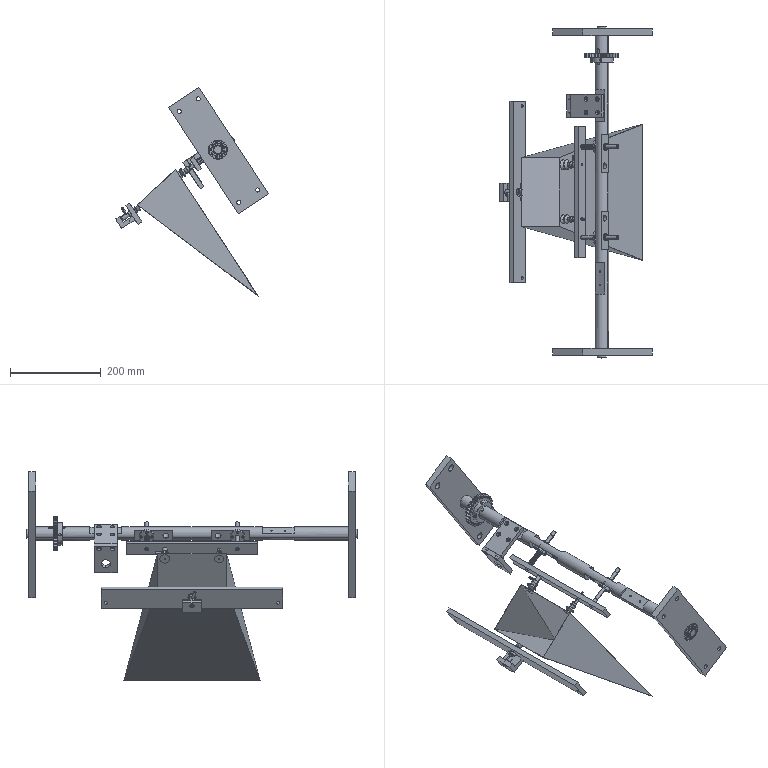Assembly | SolidWorks | mm | 20 component files | 20 solids | 970 faces | box 336.91 x 732 x 460.64 mm | volume 1533403 mm3 | cylinder 371 | plane 217 | sphere 144 | cone 104 | torus 76 | spline 58 | commonest cylinder face diameters 2.5 x32 10 x30 63.75 x29 75 x28 15 x24 6 x19 5 x18 5.5 x18
Bill of materials:
28zGear | 1 |  | Straight-tooth spur gear with a cylindrical hub on one face, a central round bore with a single keyway, and a radial hole through the hub.
BlowOpenBag | 1 |  | Solid tapered wedge or frustum-like block with flat faces only: a rectangular end face that tapers to a narrower edge, giving trapezoidal and triangular outlines in the different views.
CylinderMountingPlate01 | 1 |  | Flat rectangular plate with one large round through hole off-center and two small through holes near one edge.
GB_T276-94DeepGrooveBallBearing6004-2Z | 2 |  | Annular body that looks like a deep-groove ball bearing: an outer ring and an inner ring with a row of balls visible in the gap between them.
HB362-65EndNotTightenedGroundFlat0.25Turns10x50 | 1 | Carbon Spring Steel Wire | Helical coil of round wire with many evenly spaced turns and open, unground-looking ends, like a compression spring.
LMF8UULinearBearing | 2 |  | Flanged cylindrical bushing: a round flange with four equally spaced through holes and a coaxial cylindrical boss with a central through bore.
GuideRod01 | 2 |  | Long slender cylindrical tube with a small coaxial through bore and slightly rounded or chamfered ends.
SuctionCup1 | 1 |  | Body of revolution with two stacked conical bellows-like flares at one end and a stepped cylindrical stem of decreasing diameters, ending in a small tube with a central bore.
SuctionCup2 | 1 |  | Body of revolution like the preceding flared part: two conical bellows-like flares, stepped cylindrical sections and a thicker cylindrical end with a small axial hole, plus a solid pin sticking out sideways near the end.
SuctionCupMountingPlate | 1 |  | Long thin flat rectangular bar with four through holes in a row along its centerline; one hole is larger than the other three.
PullSuctionCupMountingPlate | 1 |  | L-shaped angle bracket of constant thickness with one through hole in one leg and two through holes in the other leg.
ShimPlate02 | 1 |  | Flat rectangular plate with four counterbored through holes in a rectangular pattern, set off to one side of the plate.
SuctionCup3 | 1 |  | Turned body that revolves around one axis. It has a plain cylindrical section, a short step, then several frustum (cone-shaped) and disc-like sections that alternate in direction to give a stepped, waisted profile. It ends in a flat circular face with a small central hole. A slender tube with an open bore branches off the cylindrical section at an angle.
SuctionCupRotatingShaftFixingPlate | 2 | 6061 Alloy | Flat rectangular plate. It has one larger circular hole near the middle and four small round holes, two near each short end, laid out symmetrically.
SupportPlate | 1 |  | Long, thin rectangular bar or plate. It has a larger circular hole at mid-length, two smaller holes beside it that look stepped, and one small hole near each end.
SwingAxis1 | 1 | 45 | Long, slender shaft with steps along its length. Both ends step down to smaller diameters. Several sections in the middle have reduced diameters or flats, and some of those flats have small round cross-holes. Seen end-on, it shows concentric circular steps.
Mates:
1. coincident | SwingAxis1-1 face at (-28.685, 307.546, 10.43) dir (0, 1, 0) | GB_T276-94DeepGrooveBallBearing6004-2Z-1 face at (-15.235, 307.546, 10.43) dir (0, -1, 0)
2. concentric | SwingAxis1-1 face at (-28.685, 325.546, 10.43) dir (0, -1, 0) r 10 | GB_T276-94DeepGrooveBallBearing6004-2Z-1 face at (-28.685, 325.966, 10.43) dir (0, 1, 0) r 10
3. concentric | SwingAxis1-1 face at (-28.685, -406.454, 10.43) dir (0, 1, 0) r 10 | GB_T276-94DeepGrooveBallBearing6004-2Z-2 face at (-28.685, -406.875, 10.43) dir (0, -1, 0) r 10
4. coincident | SwingAxis1-1 face at (-28.685, -388.454, 10.43) dir (0, -1, 0) | GB_T276-94DeepGrooveBallBearing6004-2Z-2 face at (-42.135, -388.454, 10.43) dir (0, 1, 0)
5. concentric | SwingAxis1-1 face at (-28.685, -388.454, 10.43) dir (0, 1, 0) r 15 | 28zGear-1 face at (-28.685, 265.546, 10.43) dir (0, -1, 0) r 15
6. distance | 28zGear-1 face at (-28.685, 265.546, 10.43) dir (0, 1, 0) | SwingAxis1-1 face at (-28.685, 325.546, 10.43) dir (0, 1, 0)
7. coincident | GB_T276-94DeepGrooveBallBearing6004-2Z-1 face at (-8.285, 307.546, 10.43) dir (0, -1, 0) | SuctionCupRotatingShaftFixingPlate-1 face at (-28.685, 307.546, 10.43) dir (0, 1, 0)
8. concentric | GB_T276-94DeepGrooveBallBearing6004-2Z-1 face at (-28.685, 313.546, 10.43) dir (0, 1, 0) r 21 | SuctionCupRotatingShaftFixingPlate-1 face at (-28.685, 307.546, 10.43) dir (0, 1, 0) r 21
9. coincident | GB_T276-94DeepGrooveBallBearing6004-2Z-2 face at (-49.085, -388.454, 10.43) dir (0, 1, 0) | SuctionCupRotatingShaftFixingPlate-2 face at (-28.685, -388.454, 10.43) dir (0, -1, 0)
10. concentric | GB_T276-94DeepGrooveBallBearing6004-2Z-2 face at (-28.685, -394.454, 10.43) dir (0, -1, 0) r 21 | SuctionCupRotatingShaftFixingPlate-2 face at (-28.685, -388.454, 10.43) dir (0, -1, 0) r 21
11. coincident | SuctionCupRotatingShaftFixingPlate-1 face at (82.741, 304.546, -86.989) dir (0.8372, 0, 0.5469) | SuctionCupRotatingShaftFixingPlate-2 face at (82.741, -385.454, -86.989) dir (0.8372, 0, 0.5469)
12. angle | SwingAxis1-1 face at (-30.194, 32.046, 27.363) dir (0.8371, 0, 0.5471) | SuctionCupRotatingShaftFixingPlate-1 face at (82.741, 304.546, -86.989) dir (0.8372, 0, 0.5469)
13. concentric | SwingAxis1-1 face at (-16.128, 59.546, 18.636) dir (-0.8371, 0, -0.5471) r 7.5 | LMF8UULinearBearing-1 face at (-35.382, 59.546, 6.053) dir (0.8371, 0, 0.5471) r 7.5
14. coincident | SwingAxis1-1 face at (-43.587, 32.046, 18.61) dir (-0.8371, 0, -0.5471) | LMF8UULinearBearing-1 face at (-35.382, 59.546, 6.053) dir (0.8371, 0, 0.5471)
15. coincident | LMF8UULinearBearing-1 face at (-39.567, 59.546, 3.318) dir (-0.8371, 0, -0.5471) | LMF8UULinearBearing-2 face at (-39.567, -140.454, 3.318) dir (-0.8371, 0, -0.5471)
16. concentric | SwingAxis1-1 face at (-16.128, -140.454, 18.636) dir (-0.8371, 0, -0.5471) r 7.5 | LMF8UULinearBearing-2 face at (-35.382, -140.454, 6.053) dir (0.8371, 0, 0.5471) r 7.5
17. concentric | LMF8UULinearBearing-1 face at (-35.382, 59.546, 6.053) dir (0.8371, 0, 0.5471) r 4 | NewSuctionCupGroup-1/GuideRod01-1 face at (-73.051, 59.546, -18.564) dir (0.8371, 0, 0.5471) r 4
18. concentric | LMF8UULinearBearing-2 face at (-35.382, -140.454, 6.053) dir (0.8371, 0, 0.5471) r 4 | NewSuctionCupGroup-1/GuideRod01-2 face at (-73.051, -140.454, -18.564) dir (0.8371, 0, 0.5471) r 4
19. distance | NewSuctionCupGroup-1/SuctionCupMountingPlate-1 face at (-73.051, -40.454, -18.564) dir (0.8371, 0, 0.5471) | LMF8UULinearBearing-1 face at (-39.567, 59.546, 3.318) dir (-0.8371, 0, -0.5471)
20. coincident | BlowOpenBag-1 face at (60.974, 109.546, -313.217) dir (0.8371, 0, 0.5471) | NewSuctionCupGroup-1/SuctionCup2-1 face at (-120.077, 20.154, -36.176) dir (-0.8371, 0, -0.5471)
21. coincident | BlowOpenBag-1 edge at (-122.275, 35.546, -32.813) dir (0, -1, 0) | NewSuctionCupGroup-1/SuctionCupMountingPlate-1 face at (-81.257, 104.546, -6.008) dir (-0.5471, 0, 0.8371)
22. width | BlowOpenBag-1 face at (-122.006, -116.354, -33.247) dir (0, 1, 0) | BlowOpenBag-1 face at (-122.006, 35.446, -33.247) dir (0, -1, 0) | NewSuctionCupGroup-1/SuctionCupMountingPlate-1 face at (-81.257, 104.546, -6.008) dir (0, 1, 0) | NewSuctionCupGroup-1/SuctionCupMountingPlate-1 face at (-81.257, -185.454, -6.008) dir (0, -1, 0)
23. concentric | SupportPlate-1 face at (-220.763, -40.454, -129.432) dir (0.8371, 0, 0.5471) r 9 | SuctionCup3-1 face at (-250.899, -40.454, -149.126) dir (-0.8371, 0, -0.5471) r 5
24. concentric | SuctionCup3-1 face at (-250.899, -40.454, -149.126) dir (-0.8371, 0, -0.5471) r 5 | PullSuctionCupMountingPlate-1 face at (-250.062, -40.454, -148.579) dir (-0.8371, 0, -0.5471) r 2.75
25. coincident | SuctionCup3-1 face at (-235.939, -48.334, -151.909) dir (-0.8371, 0, -0.5471) | PullSuctionCupMountingPlate-1 face at (-245.794, -60.454, -136.83) dir (0.8371, 0, 0.5471)
26. coincident | SupportPlate-1 face at (-212.557, -40.454, -141.988) dir (-0.8371, 0, -0.5471) | PullSuctionCupMountingPlate-1 face at (-218.028, -40.454, -133.617) dir (0.8371, 0, 0.5471)
27. concentric | SupportPlate-1 face at (-205.554, -25.454, -134.425) dir (0.8371, 0, 0.5471) r 5 | PullSuctionCupMountingPlate-1 face at (-213.925, -25.454, -139.895) dir (0.8371, 0, 0.5471) r 2.1
28. coincident | NewSuctionCupGroup-1/SuctionCupMountingPlate-1 face at (-73.051, -40.454, -18.564) dir (0.8371, 0, 0.5471) | HB362-65EndNotTightenedGroundFlat0.25Turns10x50-1 face at (-73.051, 59.546, -18.564) dir (-0.8371, 0, -0.5471)
29. coincident | CylinderMountingPlate01-1 face at (-78.529, 149.546, -41.258) dir (0.8371, 0, 0.5471) | ShimPlate02-1 face at (-97.129, 174.546, -12.796) dir (-0.8371, 0, -0.5471)
30. concentric | CylinderMountingPlate01-1 face at (-102.764, 134.546, -22.452) dir (-0.8371, 0, -0.5471) r 2.75 | ShimPlate02-1 face at (-94.393, 134.546, -16.982) dir (-0.8371, 0, -0.5471) r 2.1
31. concentric | CylinderMountingPlate01-1 face at (-102.764, 164.546, -22.452) dir (-0.8371, 0, -0.5471) r 2.75 | ShimPlate02-1 face at (-94.393, 164.546, -16.982) dir (-0.8371, 0, -0.5471) r 2.1
32. coincident | SwingAxis1-1 face at (-45.618, 114.546, 8.921) dir (-0.5471, 0, 0.8371) | ShimPlate02-1 face at (-58.174, 149.546, 0.7149) dir (0.5471, 0, -0.8371)
33. concentric | SwingAxis1-1 face at (-24.308, 134.546, 3.733) dir (0.5471, 0, -0.8371) r 2.1 | ShimPlate02-1 face at (-38.532, 134.546, 25.497) dir (-0.5471, 0, 0.8371) r 5
34. concentric | NewSuctionCupGroup-1/GuideRod01-1 face at (-73.051, 59.546, -18.564) dir (0.8371, 0, 0.5471) r 4 | HB362-65EndNotTightenedGroundFlat0.25Turns10x50-1 sketch point at (-73.051, 59.546, -18.564) dir (1, 0, 0)
35. concentric | SuctionCupMountingPlate-1 face at (-50.359, -1.351, -5.528) dir (0, -1, 0) r 5 | SuctionCup2-1 face at (-50.359, 14.649, -5.528) dir (0, 1, 0) r 5
36. coincident | SuctionCupMountingPlate-1 face at (-50.359, -1.351, -5.528) dir (0, -1, 0) | SuctionCup2-1 face at (-38.78, -1.351, -15.691) dir (0, 1, 0)
37. coincident | SuctionCup1-1 face at (79.641, -43.351, -5.528) dir (0, -1, 0) | SuctionCup2-1 face at (-50.968, -43.351, 5.455) dir (0, -1, 0)
38. concentric | SuctionCupMountingPlate-1 face at (69.641, 5.649, -5.528) dir (0, 1, 0) r 3.4 | SuctionCup1-1 face at (69.641, 14.649, -5.528) dir (0, 1, 0) r 3.4
39. concentric | SuctionCupMountingPlate-1 face at (-90.359, -4.351, -5.528) dir (0, -1, 0) r 2.25 | GuideRod01-1 face at (-90.359, 5.649, -5.528) dir (0, 1, 0) r 4
40. coincident | SuctionCupMountingPlate-1 face at (9.641, 5.649, -5.528) dir (0, 1, 0) | GuideRod01-1 face at (-90.359, 5.649, -5.528) dir (0, -1, 0)
41. coincident | SuctionCupMountingPlate-1 face at (9.641, 5.649, -5.528) dir (0, 1, 0) | GuideRod01-2 face at (109.641, 5.649, -5.528) dir (0, -1, 0)
42. concentric | SuctionCupMountingPlate-1 face at (109.641, -4.351, -5.528) dir (0, -1, 0) r 2.25 | GuideRod01-2 face at (109.641, 5.649, -5.528) dir (0, 1, 0) r 4